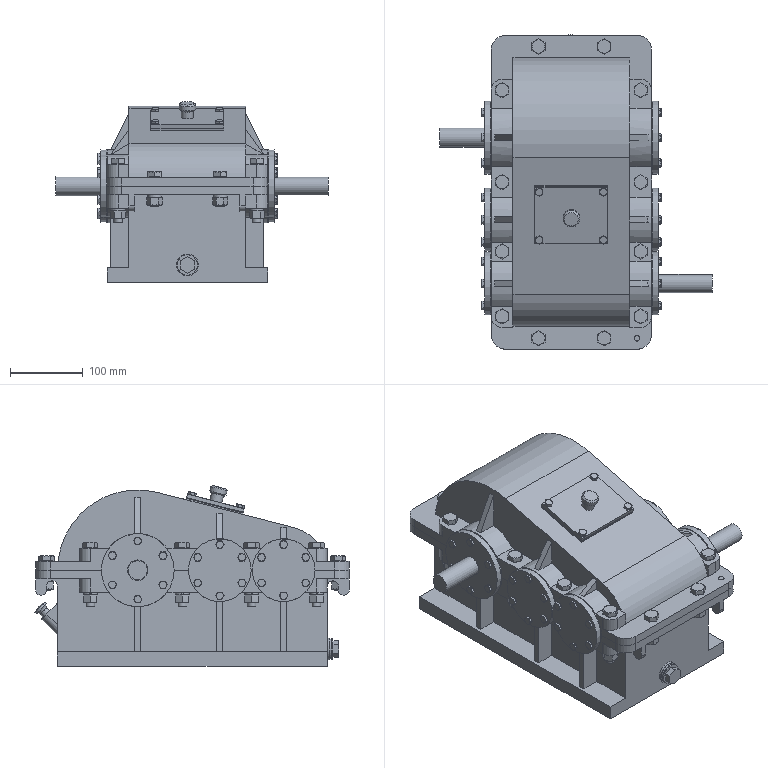Assembly | NX | mm | 125 component files | 197 solids | 3196 faces | box 373.25 x 431.26 x 247.99 mm | volume 7361855 mm3 | plane 1003 | cylinder 651 | cone 610 | spline 550 | other 250 | sphere 67 | torus 65 | commonest cylinder face diameters 6.5 x80 143.63 x60 118.63 x50 8.74 x40 5.795 x40 6 x40 68.75 x30 55 x26
Bill of materials:
unnamed part 1 | 4 |  | Thin flat annular ring with a large central opening and six small round through-holes evenly spaced on a circle.
unnamed part 2 | 1 |  | Solid stepped round shaft with several diameter steps, a raised integral collar near mid-length and one rounded-end keyway slot on the segment next to the collar.
unnamed part 3 | 1 |  | Circular flange plate with a central through-bore, six small through-holes evenly spaced on a bolt circle and a smaller-diameter raised hub on one face.
unnamed part 4 | 1 |  | Stepped shaft with an integral straight-tooth spur gear section near one end and several cylindrical journal steps of decreasing diameter toward the other end.
unnamed part 5 | 1 |  | Turned knob- or pin-like part: a large cylindrical head with a chamfered top edge, a smaller cylindrical body with a radial cross-hole, and a narrower end stem with a reduced neck or groove.
GB93-87,12 | 12 |  | Single Coil Spring Lock Washer, Normal Type, GB 93-87,12
unnamed part 6 | 1 |  | Straight-tooth spur gear with many teeth (roughly 40-50), a central bore with one keyway and a recessed annular pocket on one face around a hub area.
unnamed part 7 | 1 |  | Hex-head plug-like part with an integral round flange or collar under the hex and a plain cylindrical shank.
unnamed part 8 | 1 |  | Straight-tooth spur gear with a high tooth count (roughly 55-65), a central bore with one keyway and a recessed annular face pocket around the hub region.
unnamed part 9 | 1 |  | Wide-face straight-tooth spur gear (pinion-like) with about 30 teeth, a large central bore with one keyway and plain flat end faces.
unnamed part 10 | 1 |  | Open-top rectangular box-shaped housing with a perimeter top flange carrying bolt holes, three semicircular bore cutouts in each long wall, a wider base flange, vertical ribs below the cutouts and a small round boss with a hole on one end wall.
unnamed part 11 | 2 |  | Annular ring with a thin, larger-diameter radial flange at mid-thickness and narrower cylindrical bands on both sides of it.
unnamed part 12 | 1 |  | Solid stepped round shaft with a raised central collar, a larger-diameter journal segment on each side carrying one rounded-end keyway each, and smaller-diameter end segments.
unnamed part 13 | 1 |  | Long hollow cover with a flat rectangular base flange that has rounded corners. The shell rises from a low rounded end to a taller rounded end. Three semicircular cutouts of increasing size run along the base on each long side. There is a rectangular opening on top with four small holes around it.
GB-T292_AC-1994,7006_AC | 4 |  | Open annular rolling-element assembly shaped like a radial ball bearing: concentric outer and inner rings with a single row of spherical balls between them, no visible shields, seals, or cage.
GB-T292_AC-1994,7007_AC | 2 |  | Open annular assembly shaped like a radial ball bearing, very similar to unnamed part: outer ring, inner ring, and a single row of spherical balls with no visible shields or cage.
unnamed part 14 | 1 |  | Solid bar with flat parallel faces and fully rounded ends, like a stadium shape in plan view.
GB-T119.1-2000,8x24 | 1 |  | Parallel Pin, GB-T 119.1-2000,8x24
GB-T848-2002,M16 | 1 |  | Thin, flat annular ring like a plain washer or spacer, with a circular outer edge, a concentric circular through-hole, and a uniform rectangular cross-section.
unnamed part 15 | 2 |  | Solid bar with flat parallel faces and rounded ends in plan view, similar in form to unnamed part 14.
unnamed part 16 | 1 |  | Round stepped pin with a wide disc-shaped head and a curved (filleted or flared) underside. Below the head are two shorter stepped diameters, then a long thin straight shank.
unnamed part 17 | 1 |  | Circular disc with six through holes evenly spaced on a bolt circle. A smaller, thinner concentric round boss sits on one face. There is no central bore.
unnamed part 18 | 2 |  | Very thin flat ring with a large central opening and six small holes evenly spaced around it.
GB-T6170_F-2000,M12x1.75 | 12 |  | Hexagonal prism with a plain round through bore and chamfered corners on both end faces.
unnamed part 19 | 1 |  | Round flange with six through holes evenly spaced and a concentric raised hub on one face. It has a central through bore with a larger stepped counterbore or recess around it.
GB-T5782-2000,M6x12 | 4 |  | Hexagon Head Bolt, GB-T 5782-2000,M6x12
unnamed part 20 | 4 |  | Plain thin ring with a rectangular cross-section and a large central opening.
GB-T5782-2000,M12x40 | 4 |  | Hexagon Head Bolt, GB-T 5782-2000,M12x40
unnamed part 21 | 4 |  | Ring-shaped bushing with a central bore and a raised outer collar around the middle of its width, giving a stepped outer surface on both sides.
GB-T5782-2000,M12x80 | 8 |  | Hexagon Head Bolt, GB-T 5782-2000,M12x80
unnamed part 22 | 1 |  | Flat rectangular plate with four through holes near the corners and one larger central through hole.
GB-T5782-2000,M6x16 | 36 |  | Hexagon Head Bolt, GB-T 5782-2000,M6x16
unnamed part 23 | 1 |  | Plain cylindrical sleeve or spacer ring with a concentric through bore and flat parallel end faces.
unnamed part 24 | 1 |  | Thin flat rectangular frame plate with a large rectangular central cutout and four round through-holes, one near each corner.
unnamed part 25 | 2 |  | Thin flat circular ring (annulus) with a rectangular cross-section and a large central opening.
unnamed part 26 | 3 |  | Solid circular disc with a smaller coaxial raised boss on one face and six evenly spaced round through-holes on a bolt circle in the outer flange area.
Mates:
1. fix | xiangti 1 component
2. touch align | shuruzhou 1 face | xiangti 1 face
3. touch align | chuandongzhoudachilun 1 face | xiangti 1 face
4. touch align | chuandongzhouxiaochilun 1 face | xiangti 1 face
5. touch align | shuchuzhoudachilun 1 face | xiangti 1 face
6. distance | chuandongzhouxiaochilun 1 face | chuandongzhoudachilun 1 face
7. distance | chuandongzhoudachilun 1 face | shuruzhou 1 face
8. distance | shuchuzhoudachilun 1 face | chuandongzhouxiaochilun 1 face
9. center | chuandongzhouxiaochilun 1 face | shuruzhou 1 face | xiangti 1 face | xiangti 1 face
10. touch align | chuandongzhou 1 face | xiangti 1 face
11. touch align | chuandongzhou 1 face | chuandongzhoudachilun 1 face
12. concentric | xiaodangyouhuan 4 | shuruzhou 1 edge
13. concentric | xiaodangyouhuan 3 edge | chuandongzhou 1 edge
14. concentric | xiaodangyouhuan 1 | shuruzhou 1 edge
15. concentric | xiaodangyouhuan 2 | chuandongzhou 1 edge
16. concentric | GB-T292_AC-1994_7006_AC 4 | xiaodangyouhuan 4
17. concentric | GB-T292_AC-1994_7006_AC 3 edge | xiaodangyouhuan 3 edge
18. concentric | GB-T292_AC-1994_7006_AC 2 | xiaodangyouhuan 2
19. concentric | GB-T292_AC-1994_7006_AC 1 | xiaodangyouhuan 1
20. touch align | shuchuzhou 1 face | shuchuzhoudachilun 1 face
21. touch align | shuchuzhou 1 face | xiangti 1 face
22. concentric | chentao 1 | shuchuzhou 1 edge
23. concentric | dadangyouhuan 2 | chentao 1
24. concentric | GB-T292_AC-1994_7007_AC 2 | dadangyouhuan 2
25. concentric | dadangyouhuan 1 | shuchuzhou 1 edge
26. concentric | GB-T292_AC-1994_7007_AC 1 | dadangyouhuan 1
27. touch align | xiaoduanmengai 3 face | xiangti 1 face
28. distance | xiaoduanmengai 3 face | xiangti 1 face
29. concentric | xiaotiaozhenghuan 4 edge | xiaoduanmengai 3 edge
30. concentric | xiaotiaozhenghuan 3 | xiaoduanmengai 2 edge
31. concentric | xiaodianpian 3 edge | xiangti 1 edge
32. concentric | xiaoduanmengai 2 edge | xiaodianpian 3 edge
33. concentric | xiaodianpian 2 edge | xiangti 1 edge
34. concentric | xiaoduanmengai 1 edge | xiaodianpian 2 edge
35. concentric | xiaotiaozhenghuan 2 | xiaoduanmengai 1 edge
36. concentric | xiaodianpian 1 edge | xiaoduantougai 1 edge
37. concentric | xiaodianpian 1 edge | xiangti 1 edge
38. concentric | xiaotiaozhenghuan 1 | xiaoduantougai 1 edge
39. touch align | daduanmengai 1 face | xiangti 1 face
40. concentric | dadianpian 2 edge | daduanmengai 1 edge
41. concentric | dadianpian 2 edge | xiangti 1 edge
42. concentric | datiaozhenghuan 2 | daduanmengai 1 edge
43. concentric | dadianpian 1 edge | daduantougai 1 edge
44. concentric | dadianpian 1 edge | xiangti 1 edge
45. concentric | datiaozhenghuan 1 | daduantougai 1 edge
46. concentric | xianggai 1 edge | xiangti 1 edge
47. concentric | pingjian8 2 | chuandongzhou 1 edge
48. concentric | pingjian10 1 | shuchuzhou 1 edge
49. concentric | pingjian8 1 | chuandongzhou 1 edge
50. concentric | youbiao 1 | xiangti 1 edge
51. concentric | luosai 1 | GB-T848-2002_M16 1
52. concentric | dianpian 1 | shikonggai 1
53. concentric | dianpian 1 | xianggai 1 arc
54. concentric | tongqisai 1 | shikonggai 1
55. concentric | GB93-87_12 1 | xiangti 1 edge
56. concentric | GB93-87_12 2 | xiangti 1 edge
57. concentric | GB93-87_12 3 | xiangti 1 edge
58. concentric | GB93-87_12 4 | xiangti 1 edge
59. concentric | GB93-87_12 11 | xiangti 1 edge
60. concentric | GB93-87_12 12 | xiangti 1 edge
61. concentric | GB93-87_12 10 | xiangti 1 edge
62. concentric | GB93-87_12 9 | xiangti 1 edge
63. concentric | GB93-87_12 8 | xiangti 1 edge
64. concentric | GB93-87_12 7 | xiangti 1 edge
65. concentric | GB93-87_12 6 | xiangti 1 edge
66. concentric | GB93-87_12 5 | xiangti 1 edge
67. concentric | GB-T6170_F-2000_M12x1_75 1 | GB93-87_12 7
68. concentric | GB-T6170_F-2000_M12x1_75 2 | GB93-87_12 8
69. concentric | GB-T6170_F-2000_M12x1_75 3 | GB93-87_12 9
70. concentric | GB-T6170_F-2000_M12x1_75 4 | GB93-87_12 10
71. concentric | GB-T6170_F-2000_M12x1_75 5 | GB93-87_12 12
72. concentric | GB-T6170_F-2000_M12x1_75 6 | GB93-87_12 11
73. concentric | GB-T6170_F-2000_M12x1_75 7 | GB93-87_12 4
74. concentric | GB-T6170_F-2000_M12x1_75 8 | GB93-87_12 3
75. concentric | GB-T6170_F-2000_M12x1_75 9 | GB93-87_12 2
76. concentric | GB-T6170_F-2000_M12x1_75 10 | GB93-87_12 1
77. concentric | GB-T6170_F-2000_M12x1_75 11 | GB93-87_12 5
78. concentric | GB-T6170_F-2000_M12x1_75 12 | GB93-87_12 6